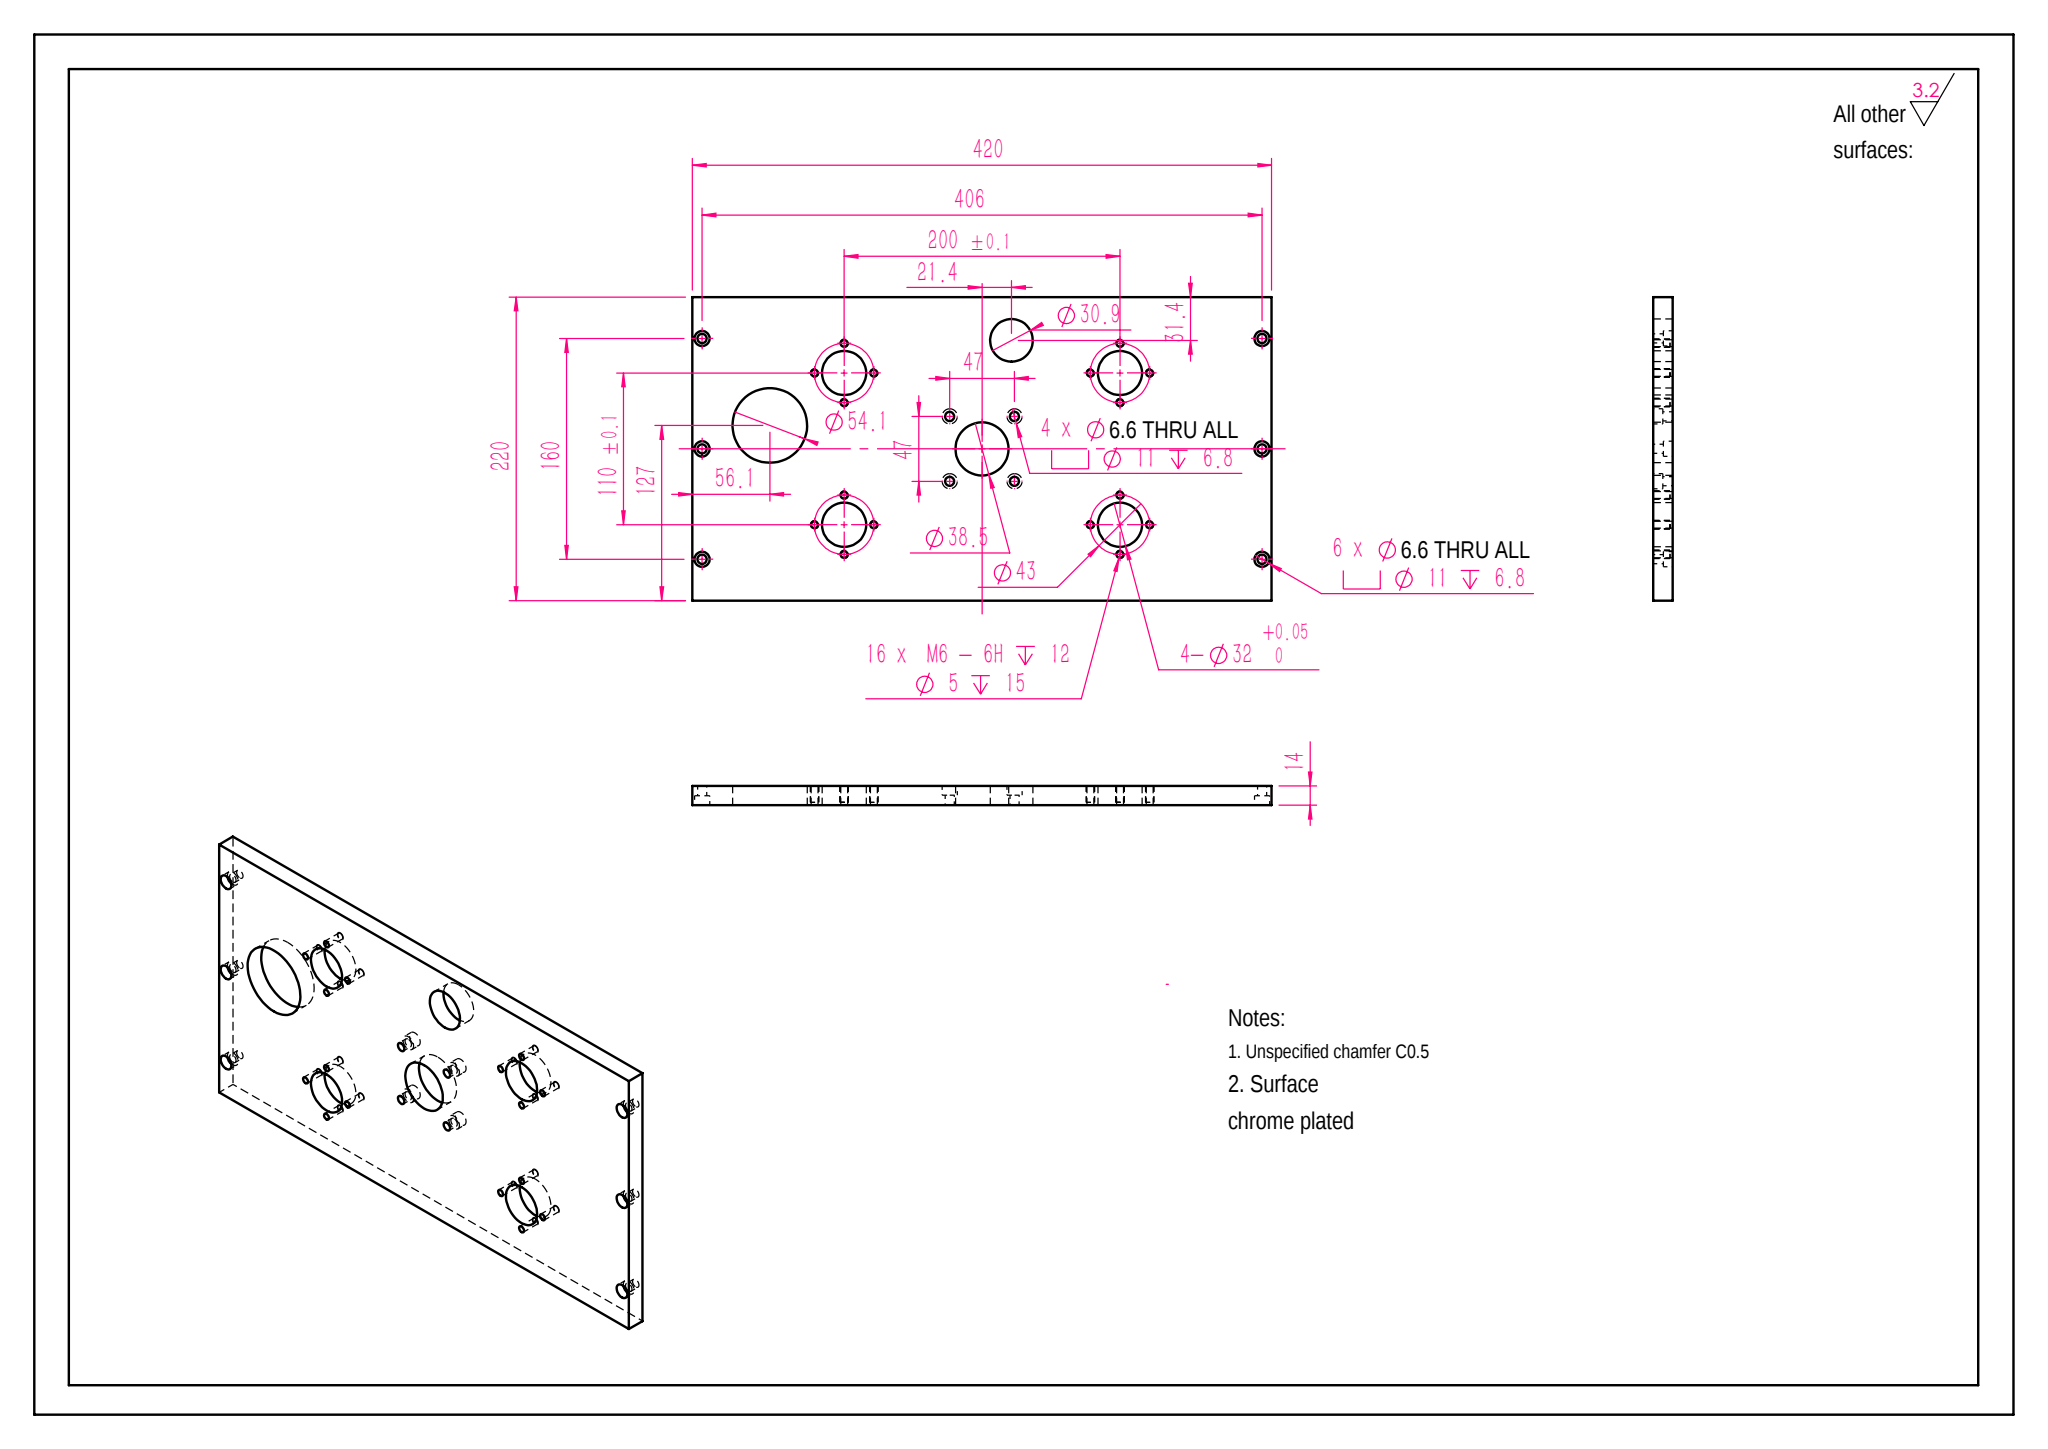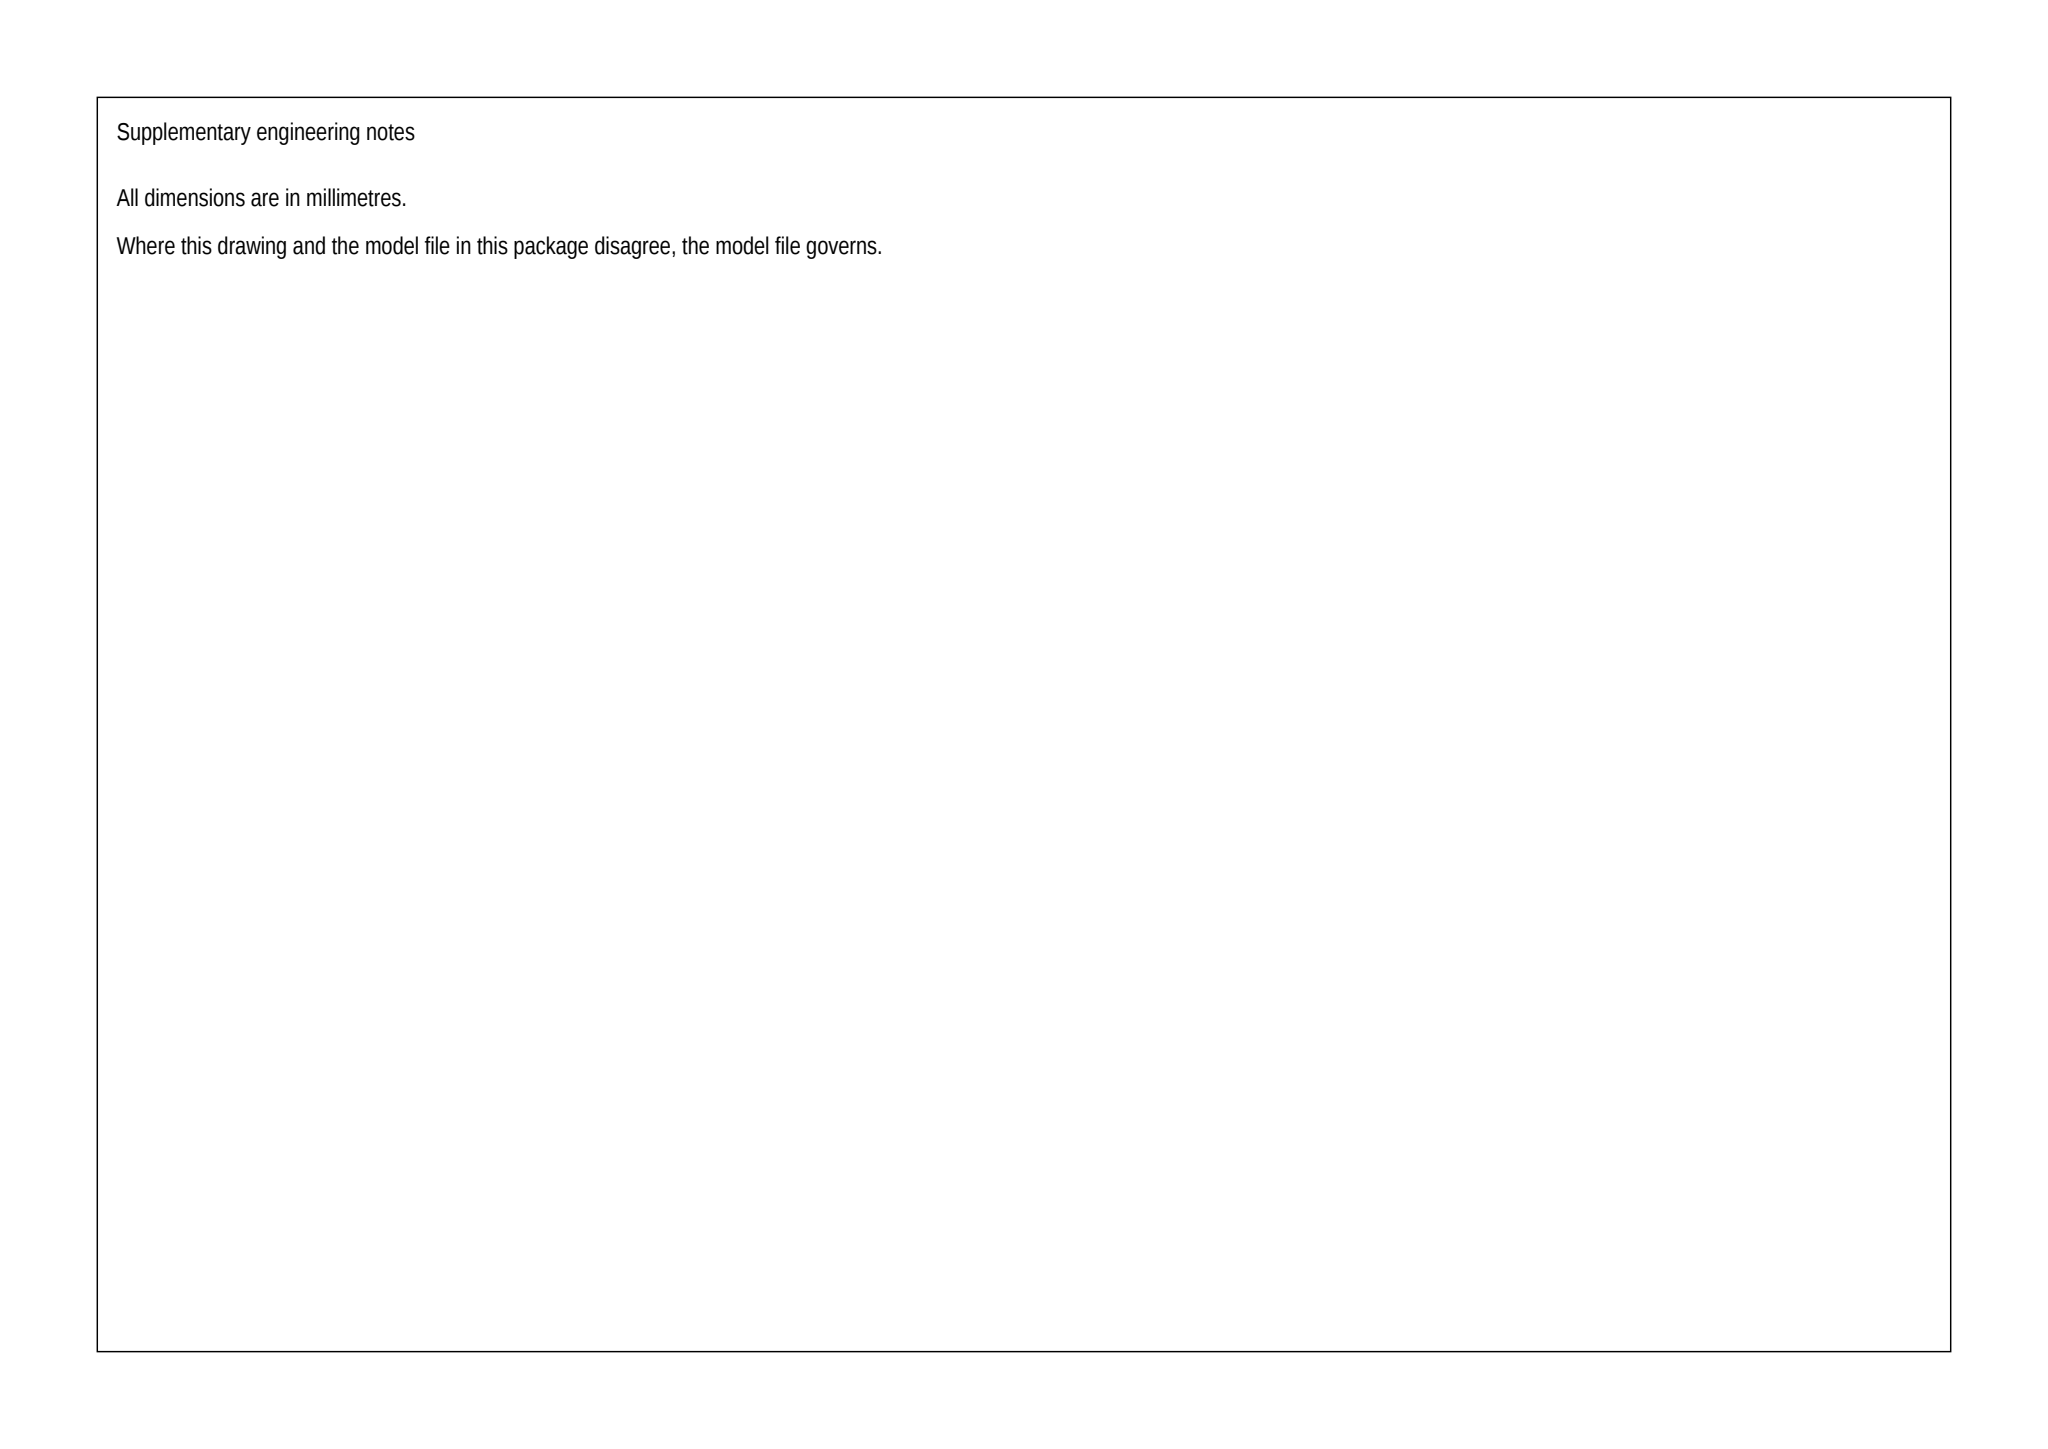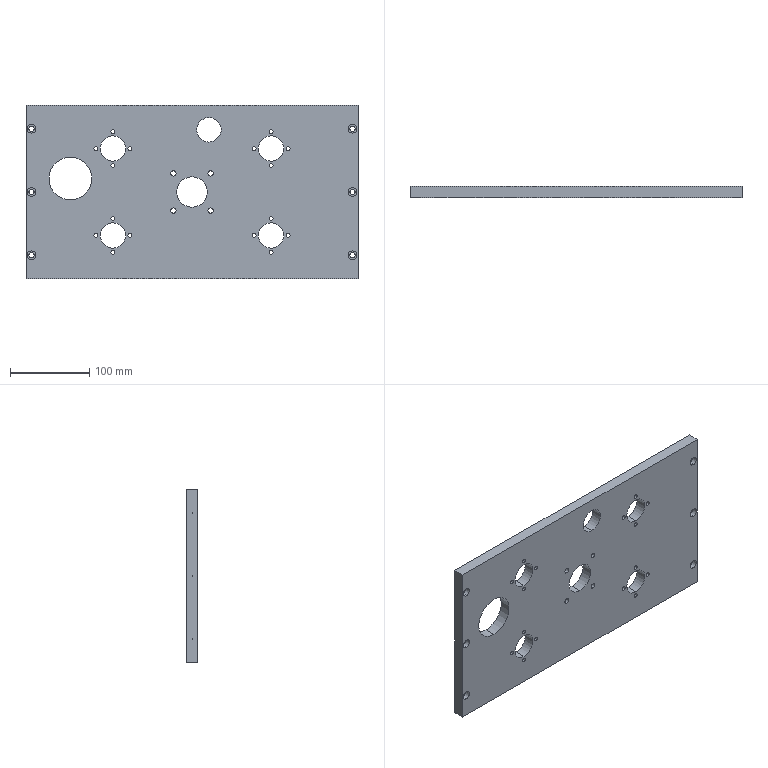Part | SolidWorks | mm | 1 solid | 102 faces | box 420 x 14 x 220 mm | volume 1176263 mm3 | cylinder 86 | plane 16 | commonest cylinder face diameters 5 x32 11 x20 6.6 x20 32 x8 54.1 x2 30.896 x2 38.5 x2
build123d program:
from build123d import *

# Parameters (mm, degrees)
SKETCH1_W                                            = 420
SKETCH1_H                                            = 220
BOSS_EXTRUDE1_DEPTH                                  = 14
SKETCH2_R                                            = 16
CUT_EXTRUDE1_DEPTH                                   = 238.478
M6_TAPPED_HOLE1_D                                    = 5
M6_TAPPED_HOLE1_DEPTH                                = 15
M6_TAPPED_HOLE1_TIP                                  = 1.502
SKETCH5_R                                            = 19.25
CUT_EXTRUDE2_DEPTH                                   = 238.478
HOLE_SIZE_ACCORDING_TO_HEX_SOCKET_HEAD_C_D           = 6.6
HOLE_SIZE_ACCORDING_TO_HEX_SOCKET_HEAD_C_CBORE_D     = 11
HOLE_SIZE_ACCORDING_TO_HEX_SOCKET_HEAD_C_CBORE_DEPTH = 6.8
HOLE_SIZE_ACCORDING_TO_HEX_SOCKET_HE_2_D             = 6.6
HOLE_SIZE_ACCORDING_TO_HEX_SOCKET_HE_2_CBORE_D       = 11
HOLE_SIZE_ACCORDING_TO_HEX_SOCKET_HE_2_CBORE_DEPTH   = 6.8
SKETCH15_R                                           = 27.05
SKETCH15_R_2                                         = 15.448
CUT_EXTRUDE3_DEPTH                                   = 80


with BuildPart() as part:
    # Sketch1 → Boss-Extrude1 (new body)
    with BuildSketch(Plane(origin=(0, 0, 0), x_dir=(1, 0, 0), z_dir=(0, 1, 0))):
        Rectangle(SKETCH1_W, SKETCH1_H)
    extrude(amount=BOSS_EXTRUDE1_DEPTH)

    # Sketch2 → Cut-Extrude1 (cut, through all)
    with BuildSketch(Plane(origin=(0, 14, 0), x_dir=(1, 0, 0), z_dir=(0, 1, 0))):
        with Locations(Location((-100, 55, 0), (0, 0, 270))):
            Circle(SKETCH2_R)
        with Locations(Location((100, 55, 0), (0, 0, 270))):
            Circle(SKETCH2_R)
    cut_extrude1 = extrude(amount=-CUT_EXTRUDE1_DEPTH, mode=Mode.SUBTRACT)

    # Mirror1: Cut-Extrude1 across plane
    add(cut_extrude1.mirror(Plane.XY), mode=Mode.SUBTRACT)

    # M6 Tapped Hole1
    with Locations(Plane(origin=(0, 14, 0), x_dir=(1, 0, 0), z_dir=(0, 1, 0))):
        with Locations((-100, 76.5), (-121.5, 55), (-100, 33.5), (-78.5, 55), (100, 76.5), (78.5, 55), (100, 33.5), (121.5, 55), (-121.5, -55), (-100, -33.5), (-78.5, -55), (-100, -76.5), (78.5, -55), (100, -33.5), (121.5, -55), (100, -76.5)):
            Hole(M6_TAPPED_HOLE1_D / 2, depth=M6_TAPPED_HOLE1_DEPTH)
            with Locations((0, 0, -(M6_TAPPED_HOLE1_DEPTH + M6_TAPPED_HOLE1_TIP / 2))):  # 118° drill point
                Cone(0, M6_TAPPED_HOLE1_D / 2, M6_TAPPED_HOLE1_TIP, mode=Mode.SUBTRACT)

    # Sketch5 → Cut-Extrude2 (cut, through all)
    with BuildSketch(Plane(origin=(0, 14, 0), x_dir=(1, 0, 0), z_dir=(0, 1, 0))):
        with Locations(Location((0, 0, 0), (0, 0, 270))):
            Circle(SKETCH5_R)
    extrude(amount=-CUT_EXTRUDE2_DEPTH, mode=Mode.SUBTRACT)

    # Hole Size according to Hex Socket Head C (through all)
    with Locations(Plane(origin=(0, 14, 0), x_dir=(1, 0, 0), z_dir=(0, 1, 0))):
        with Locations((23.5, 23.5), (-23.5, 23.5), (-23.5, -23.5), (23.5, -23.5)):
            CounterBoreHole(HOLE_SIZE_ACCORDING_TO_HEX_SOCKET_HEAD_C_D / 2, HOLE_SIZE_ACCORDING_TO_HEX_SOCKET_HEAD_C_CBORE_D / 2, HOLE_SIZE_ACCORDING_TO_HEX_SOCKET_HEAD_C_CBORE_DEPTH)

    # Hole Size according to Hex Socket He 2 (through all)
    with Locations(Plane(origin=(0, 0, 0), x_dir=(-1, 0, 0), z_dir=(0, -1, 0))):
        with Locations((203, -80), (203, 0), (203, 80), (-203, -80), (-203, 0), (-203, 80)):
            CounterBoreHole(HOLE_SIZE_ACCORDING_TO_HEX_SOCKET_HE_2_D / 2, HOLE_SIZE_ACCORDING_TO_HEX_SOCKET_HE_2_CBORE_D / 2, HOLE_SIZE_ACCORDING_TO_HEX_SOCKET_HE_2_CBORE_DEPTH)

    # Sketch15 → Cut-Extrude3 (cut)
    with BuildSketch(Plane(origin=(0, 14, 0), x_dir=(1, 0, 0), z_dir=(0, 1, 0))):
        with Locations(Location((-153.859, -16.988, 0), (0, 0, 270))):
            Circle(SKETCH15_R)
        with Locations(Location((21.356, -78.628, 0), (0, 0, 270))):
            Circle(SKETCH15_R_2)
    extrude(amount=-CUT_EXTRUDE3_DEPTH, mode=Mode.SUBTRACT)


solid = part.part